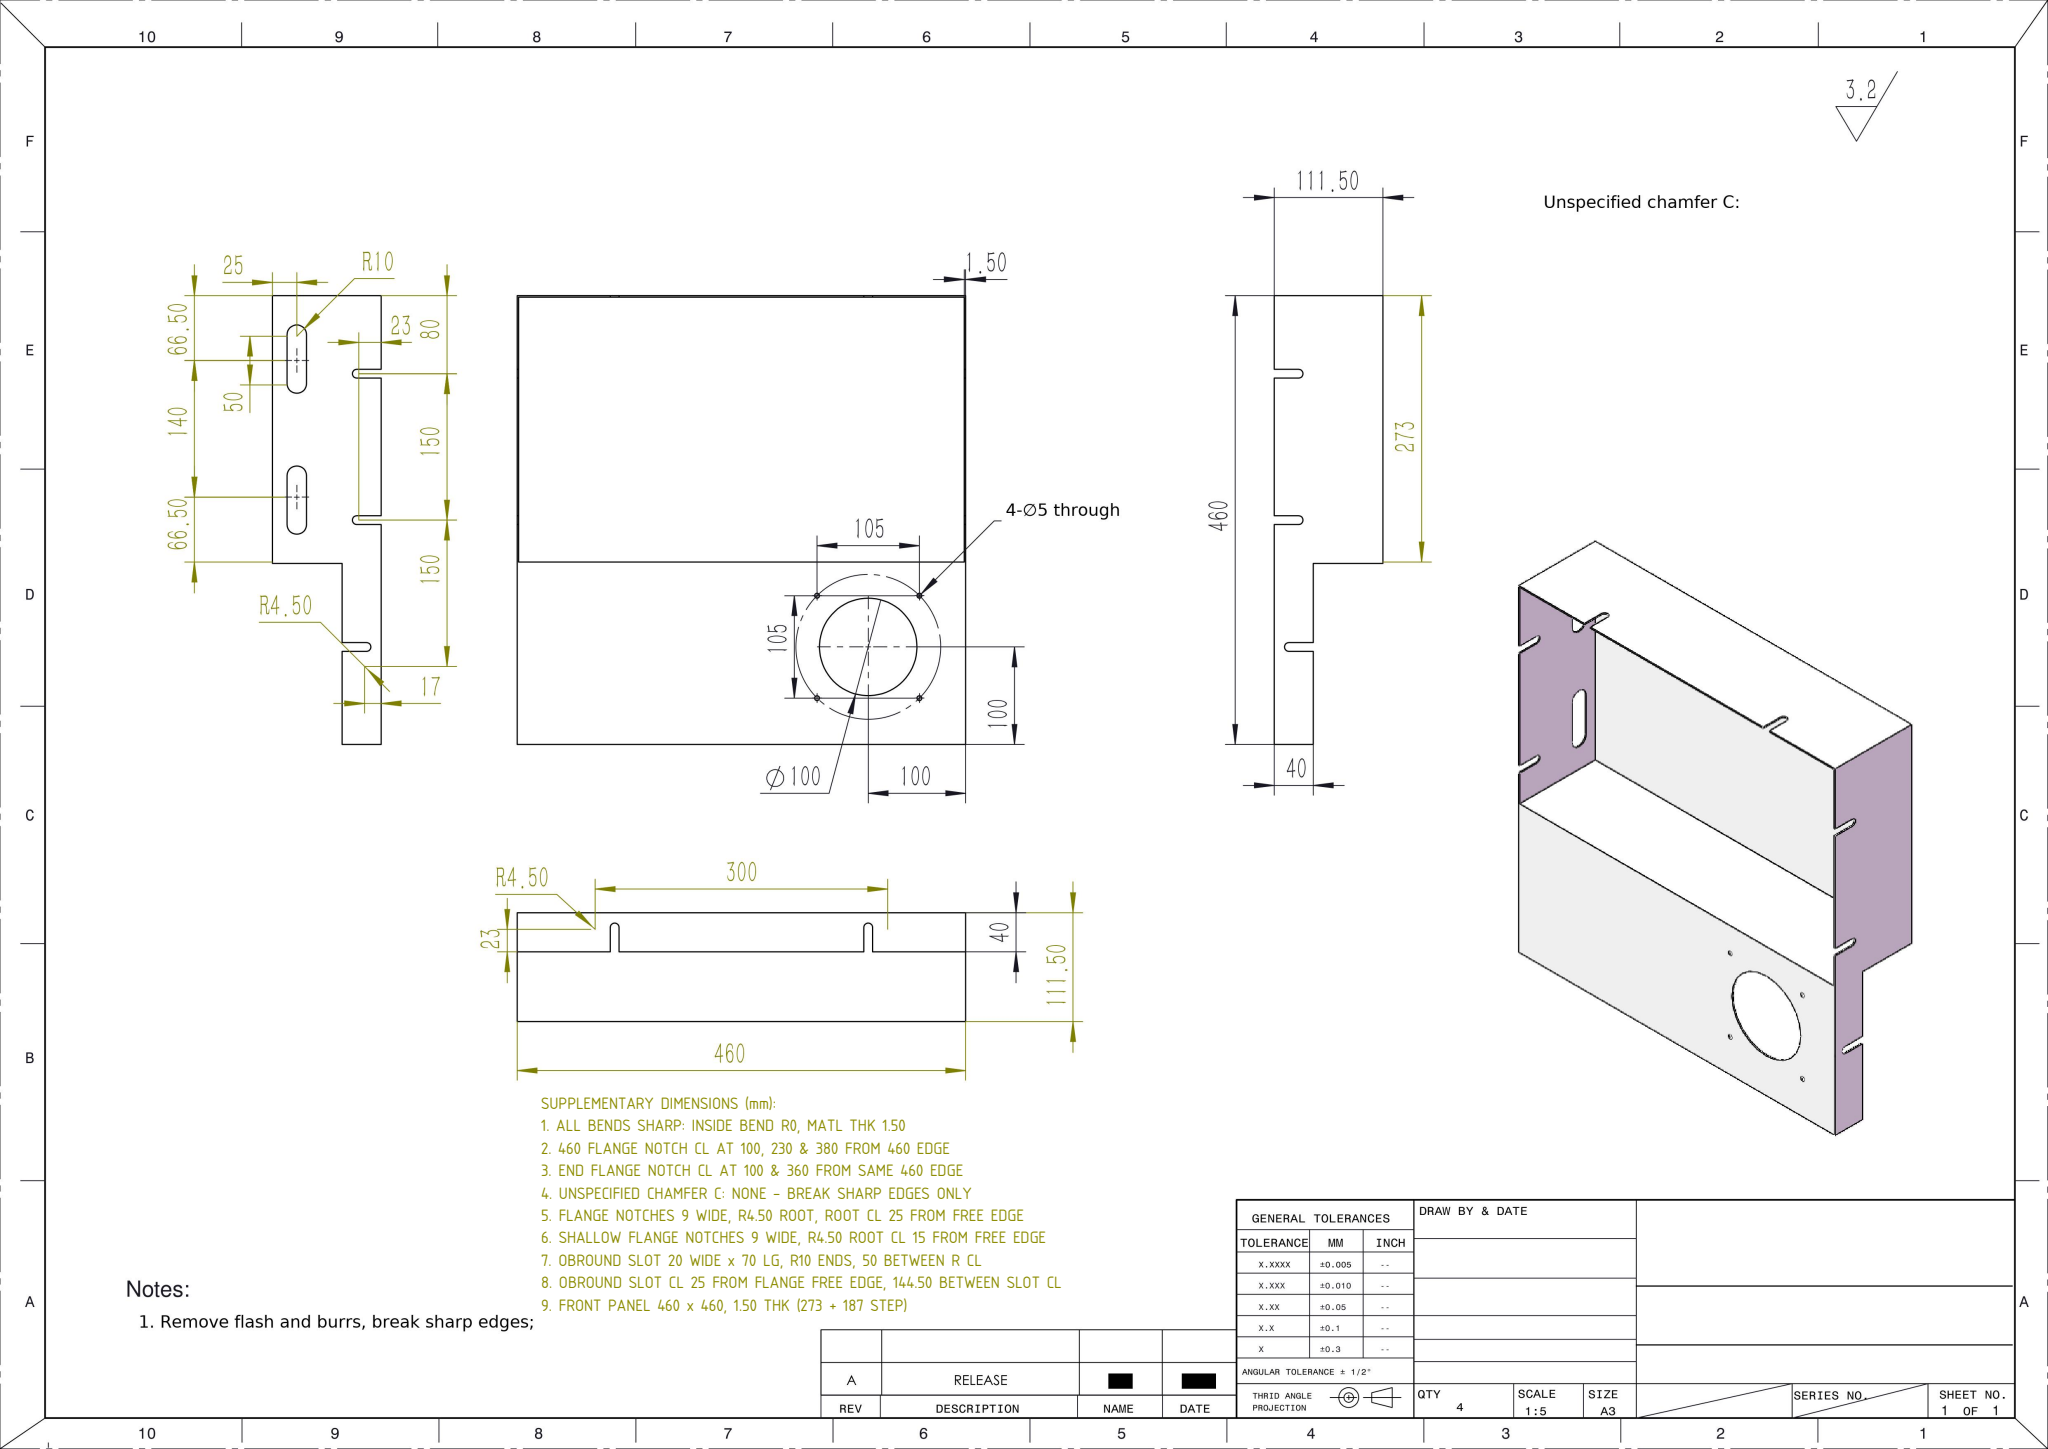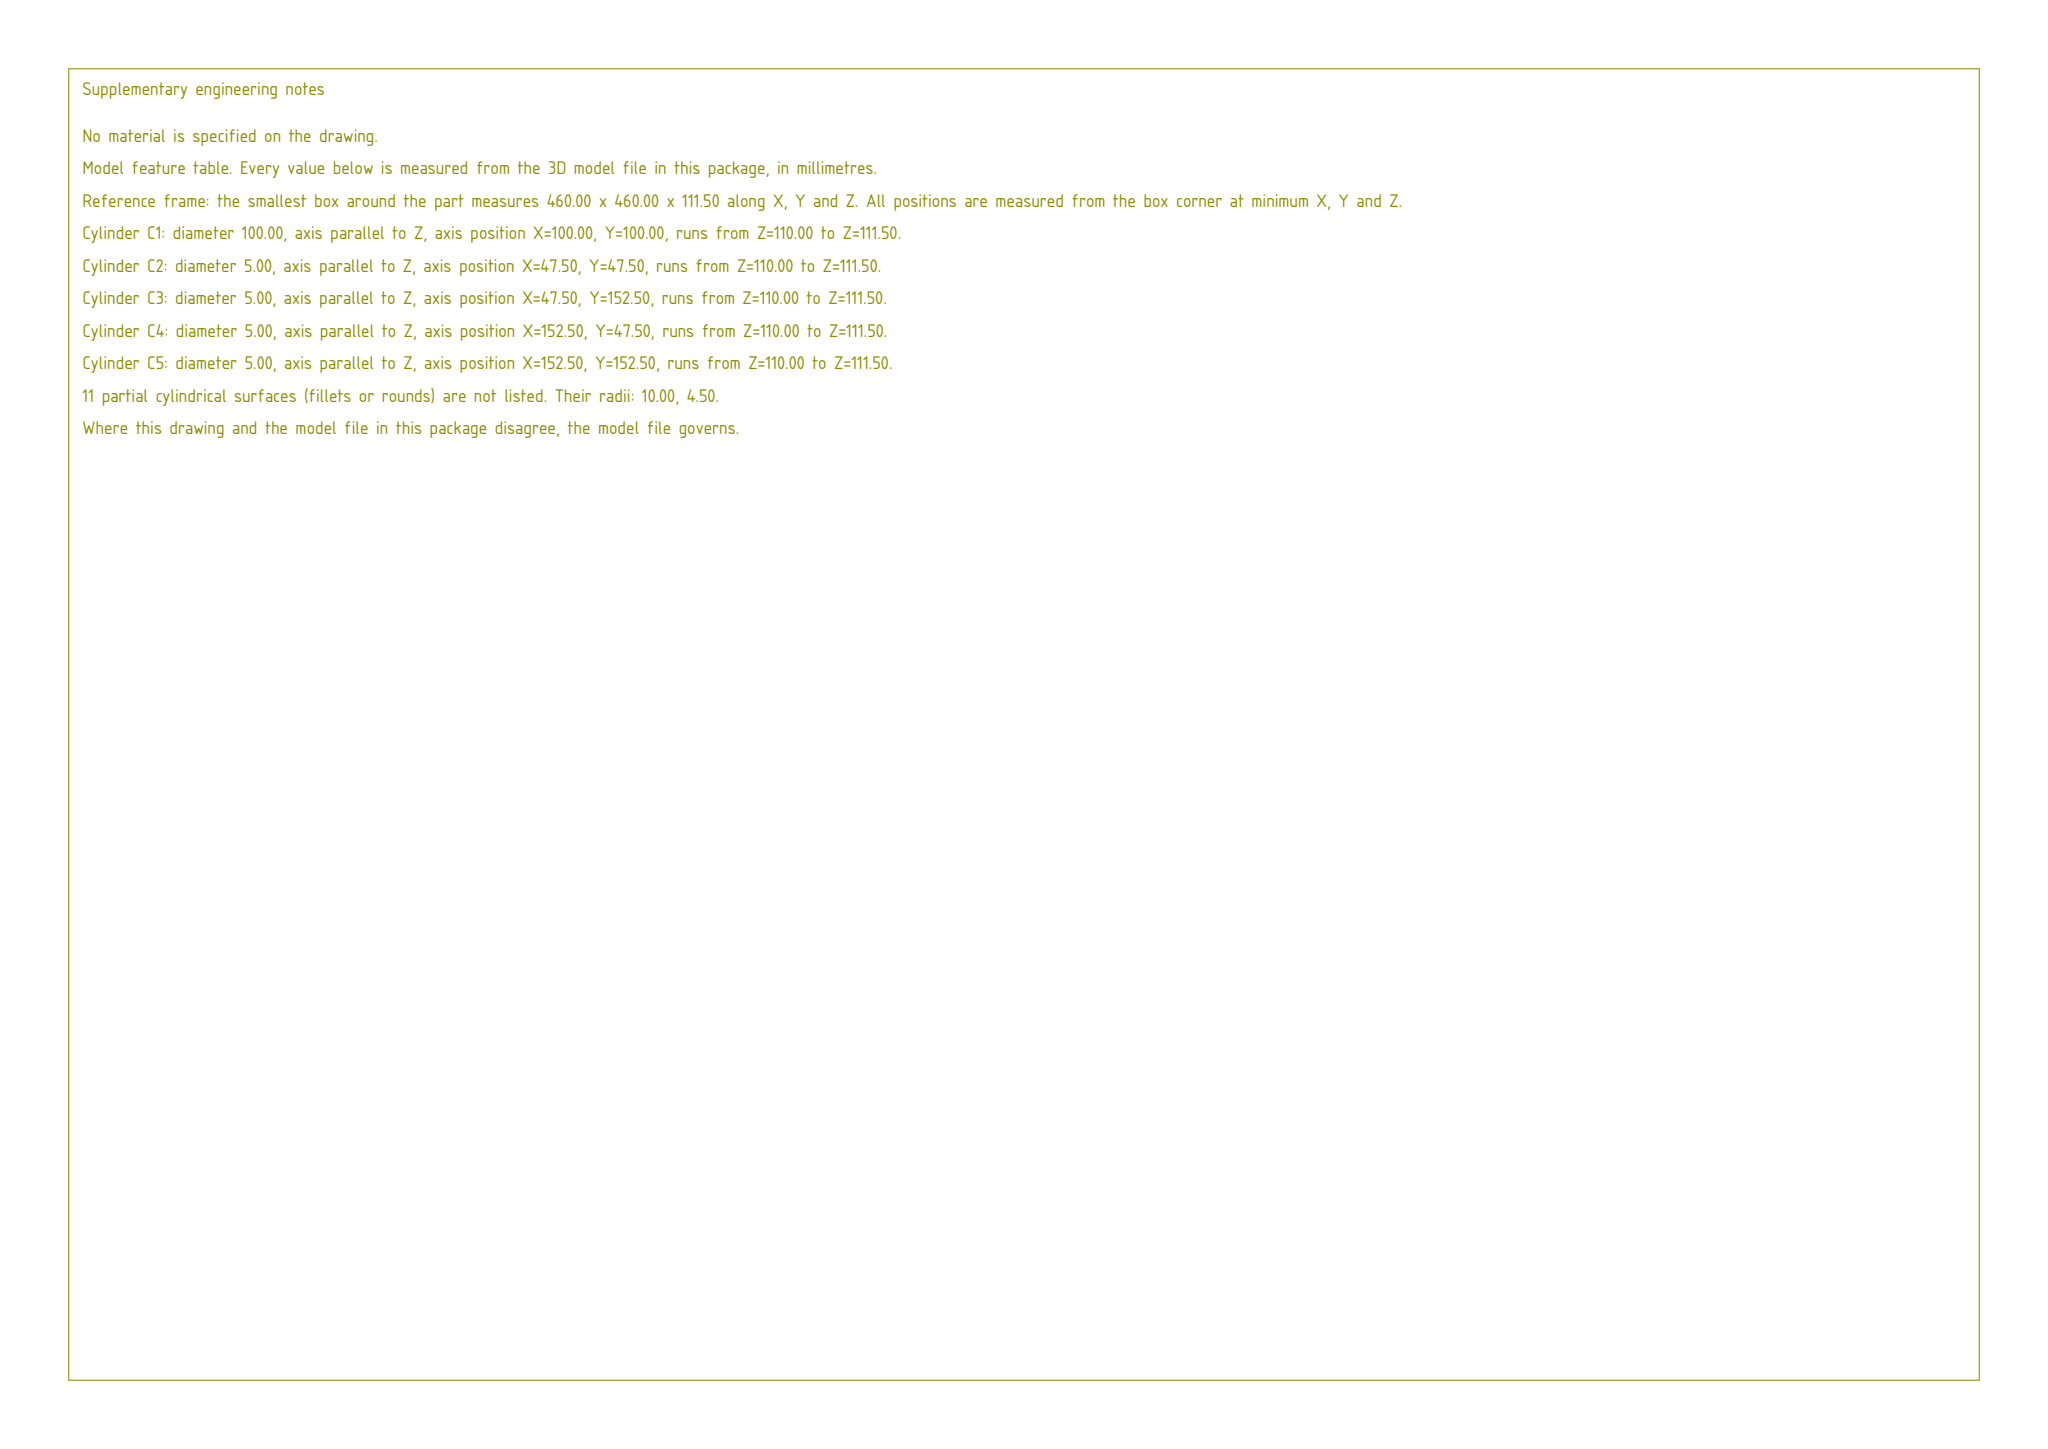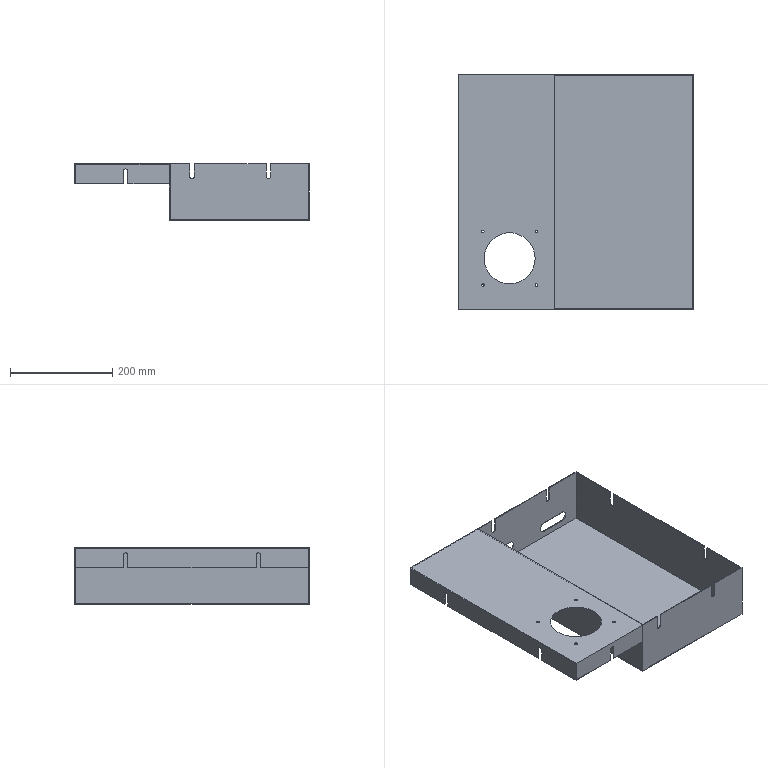Part | SolidWorks | mm | 1 solid | 79 faces | box 460 x 460 x 111.5 mm | volume 586919 mm3 | plane 50 | cylinder 29 | commonest cylinder face diameters 9 x15 5 x8 20 x4 100 x2
build123d program:
from build123d import *

# Parameters (mm, degrees)
SKETCH1_W           = 460
SKETCH1_H           = 460
BOSS_EXTRUDE1_DEPTH = 40
SHELL1_T            = -1.5
SKETCH5_R           = 50
SKETCH5_R_2         = 2.5
CUT_EXTRUDE4_DEPTH  = 975.611
SKETCH7_W           = 271.5
SKETCH7_H           = 457
CUT_EXTRUDE5_DEPTH  = 975.611
SKETCH8_W           = 274.5
SKETCH8_H           = 460
BOSS_EXTRUDE3_DEPTH = 110
SKETCH12_W          = 271.5
SKETCH12_H          = 457
CUT_EXTRUDE9_DEPTH  = 108.5
CUT_EXTRUDE7_REACH  = 994.153
CUT_EXTRUDE8_REACH  = 643.844
CUT_EXTRUDE10_REACH = 643.844
CUT_EXTRUDE11_REACH = 994.153


with BuildPart() as part:
    # Sketch1 → Boss-Extrude1 (new body)
    with BuildSketch(Plane.XY):
        with Locations((641.972, 203.51)):
            Rectangle(SKETCH1_W, SKETCH1_H)
    extrude(amount=-BOSS_EXTRUDE1_DEPTH)

    # Shell1
    shell1_openings = [part.faces().sort_by_distance(p)[0] for p in [
        (641.972, 203.51, -40),
    ]]
    offset(amount=SHELL1_T, openings=shell1_openings, kind=Kind.INTERSECTION)

    # Sketch5 → Cut-Extrude4 (cut, through all)
    with BuildSketch(Plane.XY):
        with Locations((511.972, 73.51)):
            Circle(SKETCH5_R)
        with Locations((564.472, 21.01)):
            Circle(SKETCH5_R_2)
        with Locations((564.472, 126.01)):
            Circle(SKETCH5_R_2)
        with Locations((459.472, 126.01)):
            Circle(SKETCH5_R_2)
        with Locations((459.472, 21.01)):
            Circle(SKETCH5_R_2)
    extrude(amount=-CUT_EXTRUDE4_DEPTH, mode=Mode.SUBTRACT)

    # Sketch7 → Cut-Extrude5 (cut, through all)
    with BuildSketch(Plane.XY):
        with Locations((734.722, 203.51)):
            Rectangle(SKETCH7_W, SKETCH7_H)
    extrude(amount=-CUT_EXTRUDE5_DEPTH, mode=Mode.SUBTRACT)

    # Sketch8 → Boss-Extrude3 (add)
    with BuildSketch(Plane(origin=(0, 0, -1.5), x_dir=(-1, 0, 0), z_dir=(0, 0, -1))):
        with Locations((-734.722, 203.51)):
            Rectangle(SKETCH8_W, SKETCH8_H)
    extrude(amount=BOSS_EXTRUDE3_DEPTH)

    # Sketch12 → Cut-Extrude9 (cut)
    with BuildSketch(Plane.XY.offset(-1.5)):
        with Locations((734.722, 203.51)):
            Rectangle(SKETCH12_W, SKETCH12_H)
    extrude(amount=-CUT_EXTRUDE9_DEPTH, mode=Mode.SUBTRACT)

    # Sketch10 → Cut-Extrude7 (cut, up to next)
    with BuildSketch(Plane.XZ.offset(26.49), mode=Mode.PRIVATE) as cut_extrude7_sk1:
        with BuildLine():
            Line((507.472, -45), (507.472, -15))
            ThreePointArc((507.472, -15), (511.972, -10.5), (516.472, -15))
            Line((516.472, -15), (516.472, -45))
            ThreePointArc((516.472, -45), (511.972, -49.5), (507.472, -45))
        make_face()
    cut_extrude7_tool1 = extrude(cut_extrude7_sk1.sketch, amount=-CUT_EXTRUDE7_REACH, mode=Mode.PRIVATE) & part.part
    # Sketch10 → Cut-Extrude7 (cut, up to next)
    with BuildSketch(Plane.XZ.offset(26.49), mode=Mode.PRIVATE) as cut_extrude7_sk2:
        with BuildLine():
            Line((796.472, 5), (796.472, -25))
            ThreePointArc((796.472, -25), (791.972, -29.5), (787.472, -25))
            Line((787.472, -25), (787.472, 5))
            ThreePointArc((787.472, 5), (791.972, 9.5), (796.472, 5))
        make_face()
    cut_extrude7_tool2 = extrude(cut_extrude7_sk2.sketch, amount=-CUT_EXTRUDE7_REACH, mode=Mode.PRIVATE) & part.part
    # Sketch10 → Cut-Extrude7 (cut, up to next)
    with BuildSketch(Plane.XZ.offset(26.49), mode=Mode.PRIVATE) as cut_extrude7_sk3:
        with BuildLine():
            Line((646.472, 5), (646.472, -25))
            ThreePointArc((646.472, -25), (641.972, -29.5), (637.472, -25))
            Line((637.472, -25), (637.472, 5))
            ThreePointArc((637.472, 5), (641.972, 9.5), (646.472, 5))
        make_face()
    cut_extrude7_tool3 = extrude(cut_extrude7_sk3.sketch, amount=-CUT_EXTRUDE7_REACH, mode=Mode.PRIVATE) & part.part
    cut_extrude7_1 = cut_extrude7_tool1.solids().sort_by_distance((511.972, -26.49, -30))[0]
    add(cut_extrude7_1, mode=Mode.SUBTRACT)
    cut_extrude7_2 = cut_extrude7_tool2.solids().sort_by_distance((791.972, -26.49, -10))[0]
    add(cut_extrude7_2, mode=Mode.SUBTRACT)
    cut_extrude7_3 = cut_extrude7_tool3.solids().sort_by_distance((641.972, -26.49, -10))[0]
    add(cut_extrude7_3, mode=Mode.SUBTRACT)
    cut_extrude7 = cut_extrude7_1 + cut_extrude7_2 + cut_extrude7_3  # Cut-Extrude7 as one shape, for the pattern or mirror that repeats it

    # Mirror1: Cut-Extrude7 across plane
    add(cut_extrude7.mirror(Plane(origin=(0, 203.51, 0), x_dir=(0, 0, 1), z_dir=(0, -1, 0))), mode=Mode.SUBTRACT)

    # Sketch11 → Cut-Extrude8 (cut, up to next)
    with BuildSketch(Plane.ZY.offset(-411.972), mode=Mode.PRIVATE) as cut_extrude8_sk1:
        with BuildLine():
            Line((-45, 338.01), (-15, 338.01))
            ThreePointArc((-15, 338.01), (-10.5, 333.51), (-15, 329.01))
            Line((-15, 329.01), (-45, 329.01))
            ThreePointArc((-45, 329.01), (-49.5, 333.51), (-45, 338.01))
        make_face()
    cut_extrude8_tool1 = extrude(cut_extrude8_sk1.sketch, amount=-CUT_EXTRUDE8_REACH, mode=Mode.PRIVATE) & part.part
    # Sketch11 → Cut-Extrude8 (cut, up to next)
    with BuildSketch(Plane.ZY.offset(-411.972), mode=Mode.PRIVATE) as cut_extrude8_sk2:
        with BuildLine():
            Line((-45, 69.01), (-15, 69.01))
            ThreePointArc((-15, 69.01), (-10.5, 73.51), (-15, 78.01))
            Line((-15, 78.01), (-45, 78.01))
            ThreePointArc((-45, 78.01), (-49.5, 73.51), (-45, 69.01))
        make_face()
    cut_extrude8_tool2 = extrude(cut_extrude8_sk2.sketch, amount=-CUT_EXTRUDE8_REACH, mode=Mode.PRIVATE) & part.part
    add(cut_extrude8_tool1.solids().sort_by_distance((411.972, 333.51, -30))[0], mode=Mode.SUBTRACT)
    add(cut_extrude8_tool2.solids().sort_by_distance((411.972, 73.51, -30))[0], mode=Mode.SUBTRACT)

    # Sketch13 → Cut-Extrude10 (cut, up to next)
    with BuildSketch(Plane(origin=(871.972, 0, 0), x_dir=(0, 0, -1), z_dir=(1, 0, 0)), mode=Mode.PRIVATE) as cut_extrude10_sk1:
        with BuildLine():
            Line((-5, 78.01), (25, 78.01))
            ThreePointArc((25, 78.01), (29.5, 73.51), (25, 69.01))
            Line((25, 69.01), (-5, 69.01))
            ThreePointArc((-5, 69.01), (-9.5, 73.51), (-5, 78.01))
        make_face()
    cut_extrude10_tool1 = extrude(cut_extrude10_sk1.sketch, amount=-CUT_EXTRUDE10_REACH, mode=Mode.PRIVATE) & part.part
    # Sketch13 → Cut-Extrude10 (cut, up to next)
    with BuildSketch(Plane(origin=(871.972, 0, 0), x_dir=(0, 0, -1), z_dir=(1, 0, 0)), mode=Mode.PRIVATE) as cut_extrude10_sk2:
        with BuildLine():
            Line((-5, 329.01), (25, 329.01))
            ThreePointArc((25, 329.01), (29.5, 333.51), (25, 338.01))
            Line((25, 338.01), (-5, 338.01))
            ThreePointArc((-5, 338.01), (-9.5, 333.51), (-5, 329.01))
        make_face()
    cut_extrude10_tool2 = extrude(cut_extrude10_sk2.sketch, amount=-CUT_EXTRUDE10_REACH, mode=Mode.PRIVATE) & part.part
    add(cut_extrude10_tool1.solids().sort_by_distance((871.972, 73.51, -10))[0], mode=Mode.SUBTRACT)
    add(cut_extrude10_tool2.solids().sort_by_distance((871.972, 333.51, -10))[0], mode=Mode.SUBTRACT)

    # Sketch14 → Cut-Extrude11 (cut, up to next)
    with BuildSketch(Plane(origin=(0, 433.51, 0), x_dir=(1, 0, 0), z_dir=(0, 1, 0)), mode=Mode.PRIVATE) as cut_extrude11_sk1:
        with BuildLine():
            Line((637.472, 96.5), (687.472, 96.5))
            ThreePointArc((687.472, 96.5), (697.472, 86.5), (687.472, 76.5))
            Line((687.472, 76.5), (637.472, 76.5))
            ThreePointArc((637.472, 76.5), (627.472, 86.5), (637.472, 96.5))
        make_face()
    cut_extrude11_tool1 = extrude(cut_extrude11_sk1.sketch, amount=-CUT_EXTRUDE11_REACH, mode=Mode.PRIVATE) & part.part
    # Sketch14 → Cut-Extrude11 (cut, up to next)
    with BuildSketch(Plane(origin=(0, 433.51, 0), x_dir=(1, 0, 0), z_dir=(0, 1, 0)), mode=Mode.PRIVATE) as cut_extrude11_sk2:
        with BuildLine():
            Line((781.972, 96.5), (831.972, 96.5))
            ThreePointArc((831.972, 96.5), (841.972, 86.5), (831.972, 76.5))
            Line((831.972, 76.5), (781.972, 76.5))
            ThreePointArc((781.972, 76.5), (771.972, 86.5), (781.972, 96.5))
        make_face()
    cut_extrude11_tool2 = extrude(cut_extrude11_sk2.sketch, amount=-CUT_EXTRUDE11_REACH, mode=Mode.PRIVATE) & part.part
    add(cut_extrude11_tool1.solids().sort_by_distance((662.472, 433.51, -86.5))[0], mode=Mode.SUBTRACT)
    add(cut_extrude11_tool2.solids().sort_by_distance((806.972, 433.51, -86.5))[0], mode=Mode.SUBTRACT)


solid = part.part